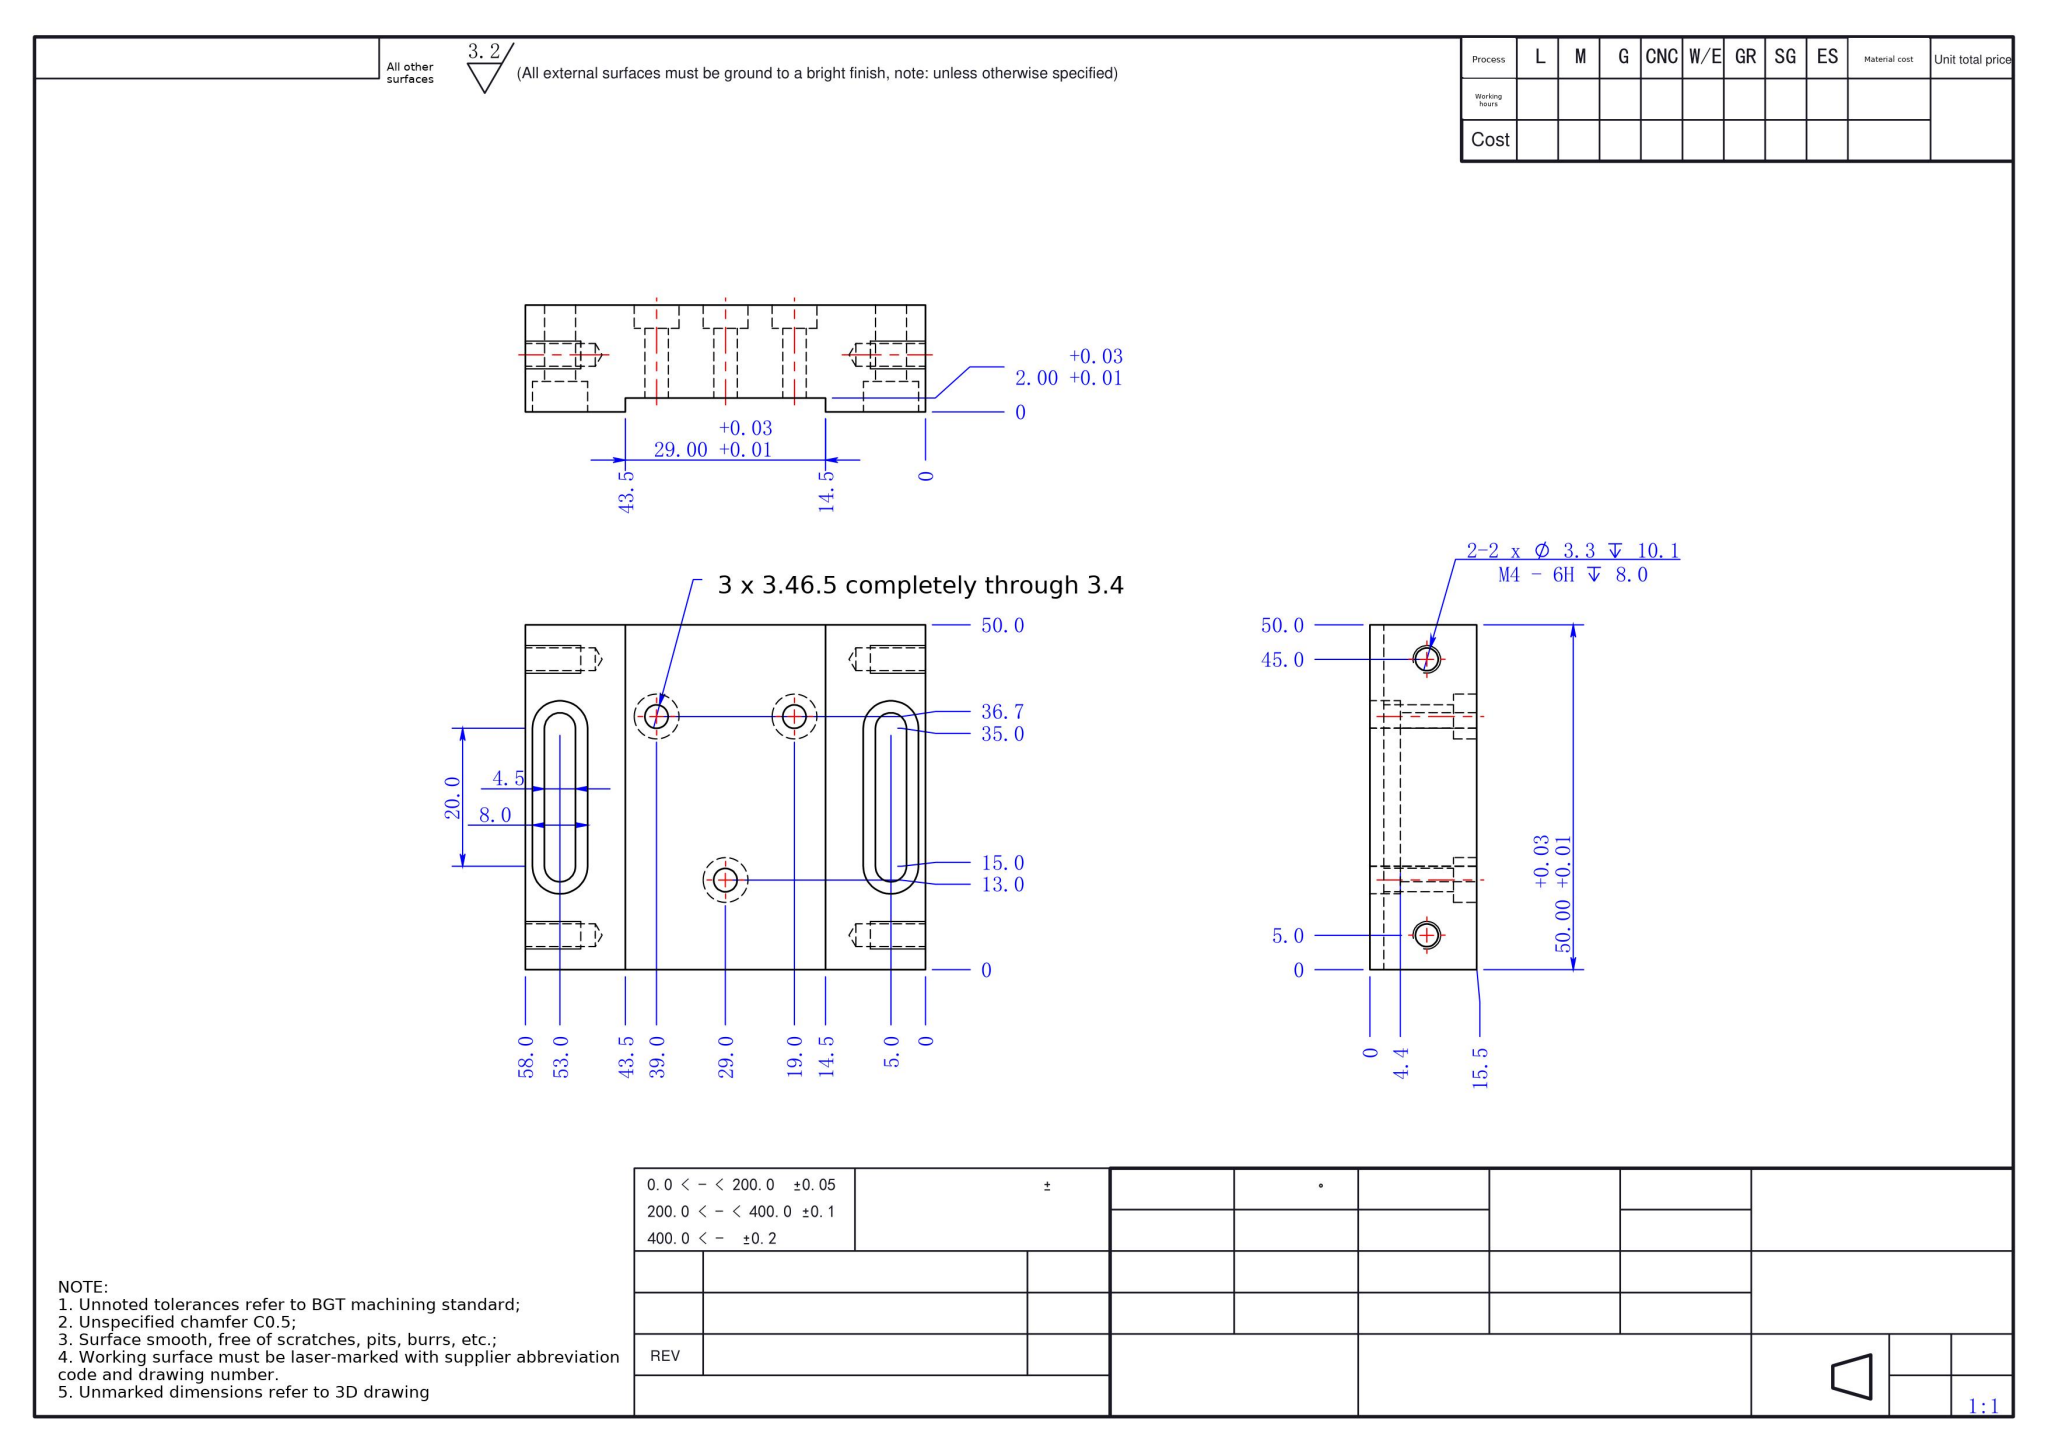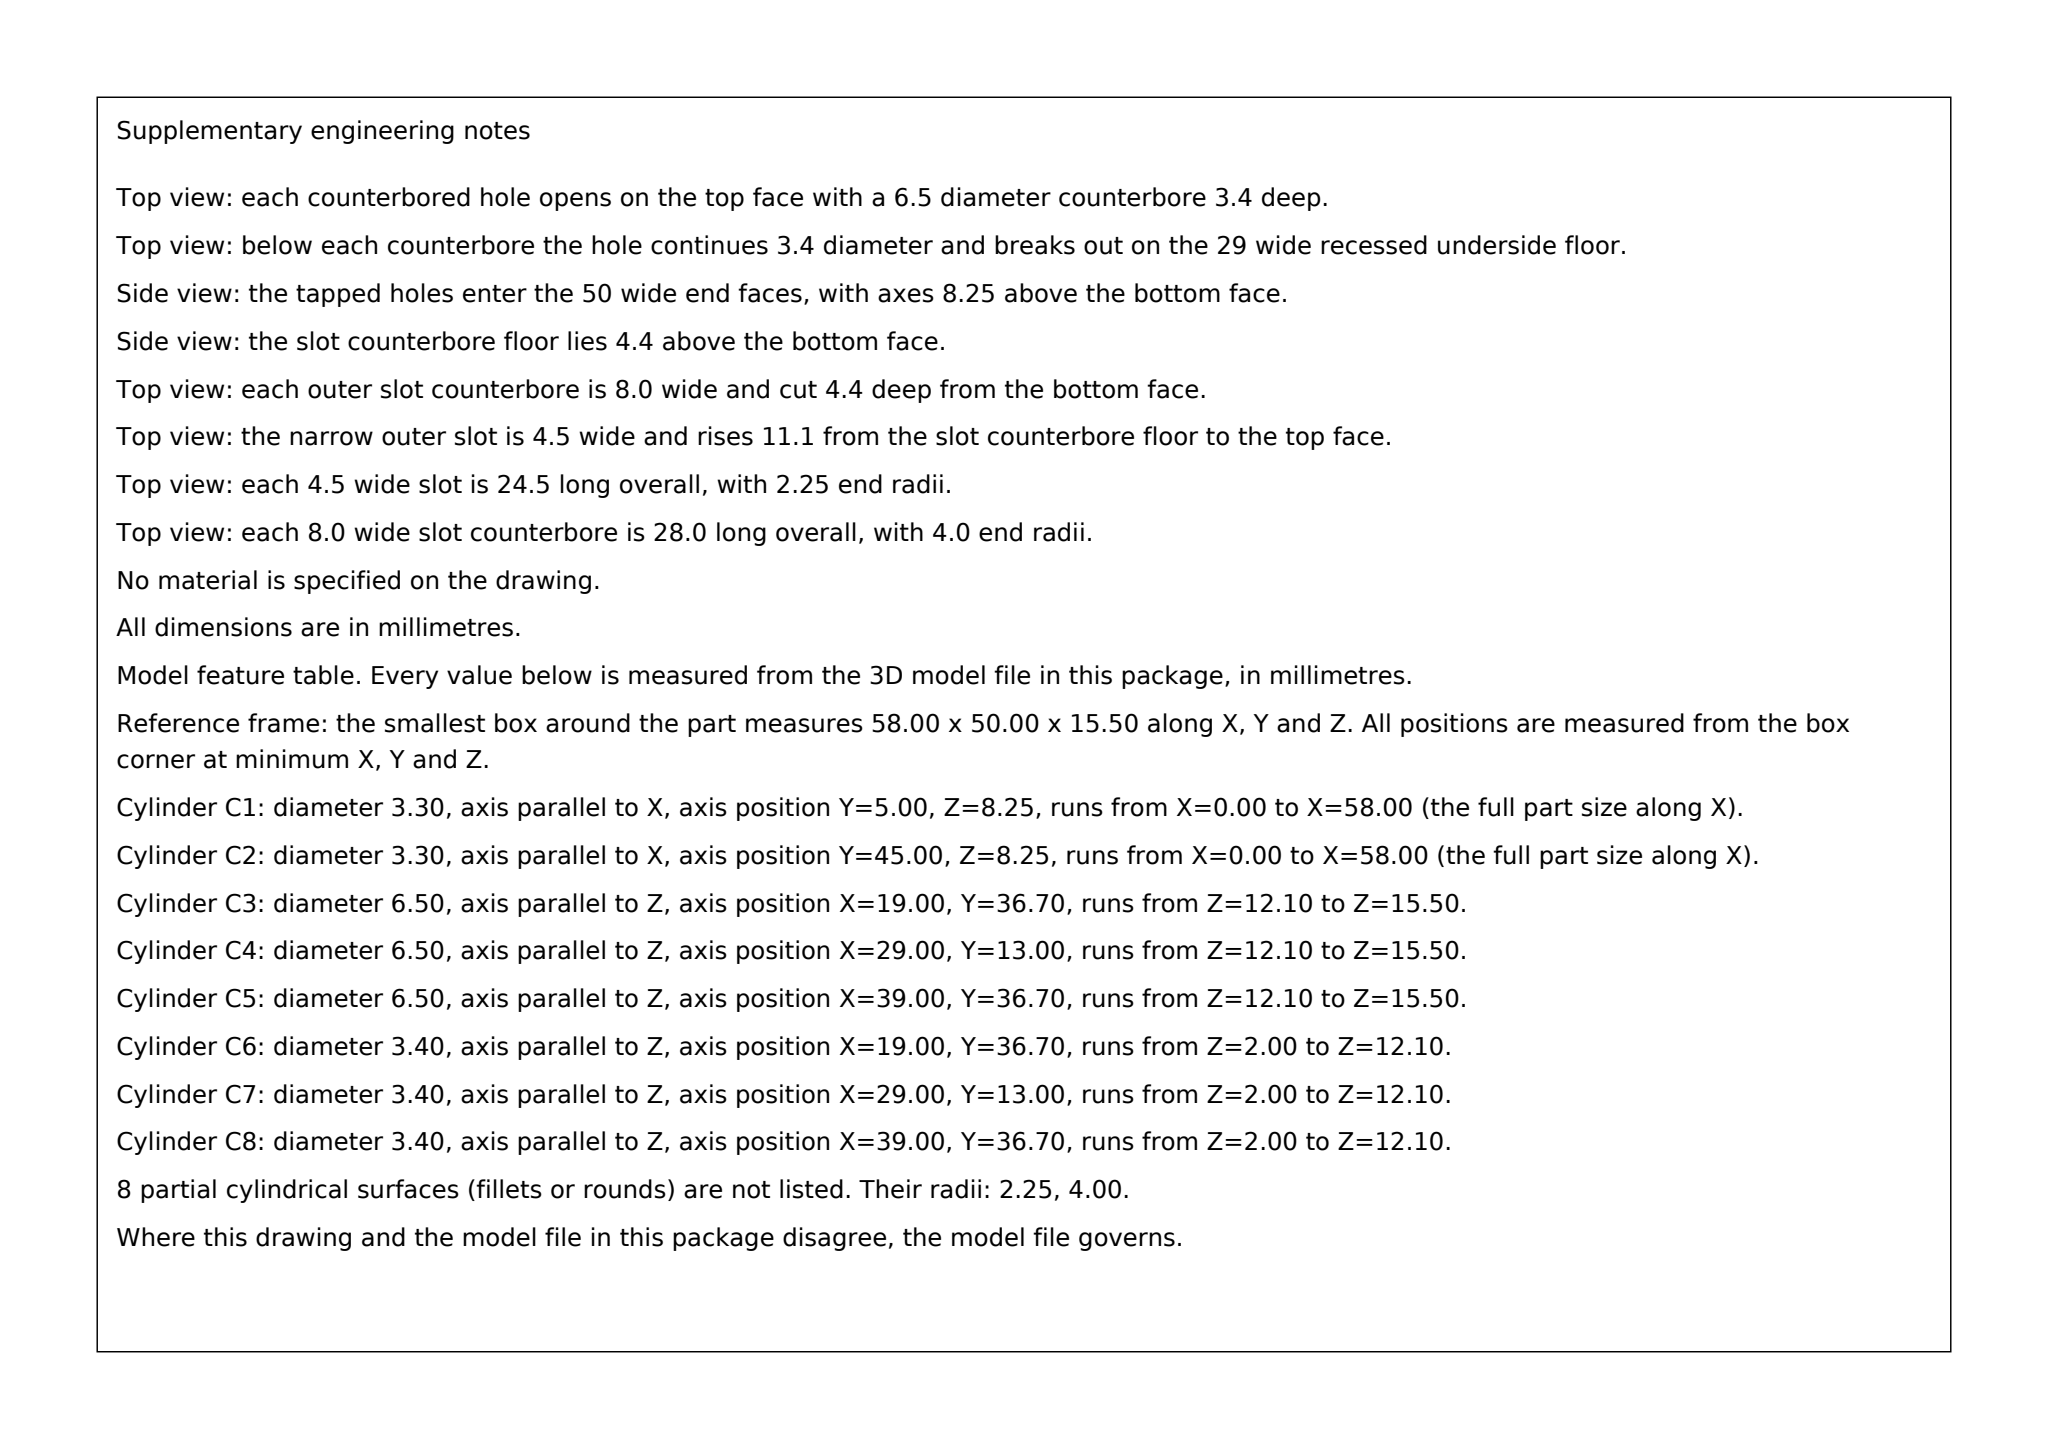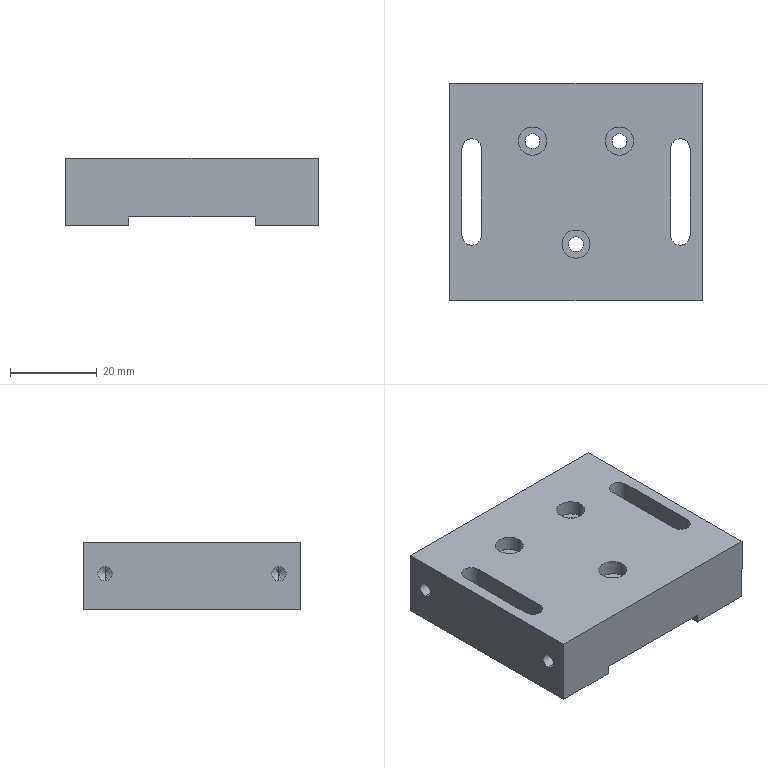Part | SolidWorks | mm | 1 solid | 59 faces | box 58 x 50 x 15.5 mm | volume 36878 mm3 | cylinder 28 | plane 23 | cone 8 | commonest cylinder face diameters 3.3 x8 6.5 x6 3.4 x6 4.5 x4 8 x4
build123d program:
from build123d import *

# Parameters (mm, degrees)
SKETCH1_W                                       = 58
SKETCH1_H                                       = 50
BOSS_EXTRUDE1_DEPTH                             = 16.5
SKETCH3_W                                       = 1
SKETCH3_H                                       = 14
CUT_EXTRUDE1_DEPTH                              = 66.278
M4_TAPPED_HOLE1_AT_2_COUNT                      = 2
M4_TAPPED_HOLE1_AT_2_PITCH                      = 40
SKETCH11_W                                      = 29
SKETCH11_H                                      = 50
CUT_EXTRUDE3_DEPTH                              = 2
M4_HEX_SOCKET_HEAD_CAP_SCREW_CBORE1_D           = 4.5
M4_HEX_SOCKET_HEAD_CAP_SCREW_CBORE1_CBORE_D     = 8
M4_HEX_SOCKET_HEAD_CAP_SCREW_CBORE1_CBORE_DEPTH = 4.4
SKETCH14_W                                      = 1
SKETCH14_H                                      = 50
CUT_EXTRUDE4_DEPTH                              = 66.278
M3_HEX_SOCKET_HEAD_CAP_SCREW_CBORE1_D           = 3.4
M3_HEX_SOCKET_HEAD_CAP_SCREW_CBORE1_CBORE_D     = 6.5
M3_HEX_SOCKET_HEAD_CAP_SCREW_CBORE1_CBORE_DEPTH = 3.4
CUT_EXTRUDE5_DEPTH                              = 42.307
CUT_EXTRUDE6_DEPTH                              = 4.4


with BuildPart() as part:
    # Sketch1 → Boss-Extrude1 (new body)
    with BuildSketch(Plane.XY):
        Rectangle(SKETCH1_W, SKETCH1_H)
    extrude(amount=BOSS_EXTRUDE1_DEPTH)

    # Sketch3 → Cut-Extrude1 (cut, through all)
    with BuildSketch(Plane(origin=(29, 0, 0), x_dir=(0, 0, -1), z_dir=(1, 0, 0))):
        with Locations((-16, 0)):
            Rectangle(SKETCH3_W, SKETCH3_H)
    extrude(amount=-CUT_EXTRUDE1_DEPTH, mode=Mode.SUBTRACT)

    # Sketch9 → M4 Tapped Hole1 (revolve, cut)
    with BuildSketch(Plane(origin=(-29, 20, 8.25), x_dir=(0, 0, 1), z_dir=(0, 1, 0))):
        Polygon((0, 0), (0, 11.091), (1.65, 10.1), (1.65, 0), align=None)
    m4_tapped_hole1 = revolve(axis=Axis((-35.35, 20, 8.25), (1, 0, 0)), mode=Mode.SUBTRACT)

    # M4 Tapped Hole1 at 2: M4 Tapped Hole1 ×2
    with Locations(*[(0, -i * M4_TAPPED_HOLE1_AT_2_PITCH, 0) for i in range(1, M4_TAPPED_HOLE1_AT_2_COUNT)]):
        add(m4_tapped_hole1, mode=Mode.SUBTRACT)

    # Mirror1: M4 Tapped Hole1 across plane
    add(m4_tapped_hole1.mirror(Plane(origin=(0, 0, 0), x_dir=(0, 0, 1), z_dir=(1, 0, 0))), mode=Mode.SUBTRACT)

    # Mirror1 copy 1 sketch → Mirror1 copy 1 (revolve, cut)
    with BuildSketch(Plane(origin=(29, -20, 8.25), x_dir=(0, 0, 1), z_dir=(0, 1, 0))):
        Polygon((0, 0), (0, -11.091), (1.65, -10.1), (1.65, 0), align=None)
    revolve(axis=Axis((35.35, -20, 8.25), (1, 0, 0)), mode=Mode.SUBTRACT)

    # Sketch11 → Cut-Extrude3 (cut)
    with BuildSketch(Plane(origin=(0, 0, 0), x_dir=(-1, 0, 0), z_dir=(0, 0, -1))):
        Rectangle(SKETCH11_W, SKETCH11_H)
    extrude(amount=-CUT_EXTRUDE3_DEPTH, mode=Mode.SUBTRACT)

    # M4 Hex Socket Head Cap Screw CBORE1 (through all)
    with Locations(Plane(origin=(0, 0, 0), x_dir=(-1, 0, 0), z_dir=(0, 0, -1))):
        with Locations((-24, 0), (24, 0)):
            CounterBoreHole(M4_HEX_SOCKET_HEAD_CAP_SCREW_CBORE1_D / 2, M4_HEX_SOCKET_HEAD_CAP_SCREW_CBORE1_CBORE_D / 2, M4_HEX_SOCKET_HEAD_CAP_SCREW_CBORE1_CBORE_DEPTH)

    # Sketch14 → Cut-Extrude4 (cut, through all)
    with BuildSketch(Plane.ZY.offset(29)):
        with Locations((16, 0)):
            Rectangle(SKETCH14_W, SKETCH14_H)
    extrude(amount=-CUT_EXTRUDE4_DEPTH, mode=Mode.SUBTRACT)

    # M3 Hex Socket Head Cap Screw CBORE1 (through all)
    with Locations(Plane.XY.offset(15.5)):
        with Locations((-10, 11.7), (10, 11.7), (0, -12)):
            CounterBoreHole(M3_HEX_SOCKET_HEAD_CAP_SCREW_CBORE1_D / 2, M3_HEX_SOCKET_HEAD_CAP_SCREW_CBORE1_CBORE_D / 2, M3_HEX_SOCKET_HEAD_CAP_SCREW_CBORE1_CBORE_DEPTH)

    # Sketch15 → Cut-Extrude5 (cut, through all)
    with BuildSketch(Plane(origin=(0, 0, 0), x_dir=(-1, 0, 0), z_dir=(0, 0, -1))):
        with BuildLine():
            Line((-26.25, -10), (-26.25, 10))
            ThreePointArc((-26.25, 10), (-24, 12.25), (-21.75, 10))
            Line((-21.75, 10), (-21.75, -10))
            ThreePointArc((-21.75, -10), (-24, -12.25), (-26.25, -10))
        make_face()
        with BuildLine():
            Line((21.75, -10), (21.75, 10))
            ThreePointArc((21.75, 10), (24, 12.25), (26.25, 10))
            Line((26.25, 10), (26.25, -10))
            ThreePointArc((26.25, -10), (24, -12.25), (21.75, -10))
        make_face()
    extrude(amount=-CUT_EXTRUDE5_DEPTH, mode=Mode.SUBTRACT)

    # Sketch16 → Cut-Extrude6 (cut)
    with BuildSketch(Plane(origin=(0, 0, 0), x_dir=(-1, 0, 0), z_dir=(0, 0, -1))):
        with BuildLine():
            Line((-28, -10), (-28, 10))
            ThreePointArc((-28, 10), (-24, 14), (-20, 10))
            Line((-20, 10), (-20, -10))
            ThreePointArc((-20, -10), (-24, -14), (-28, -10))
        make_face()
        with BuildLine():
            Line((20, -10), (20, 10))
            ThreePointArc((20, 10), (24, 14), (28, 10))
            Line((28, 10), (28, -10))
            ThreePointArc((28, -10), (24, -14), (20, -10))
        make_face()
    extrude(amount=-CUT_EXTRUDE6_DEPTH, mode=Mode.SUBTRACT)


solid = part.part